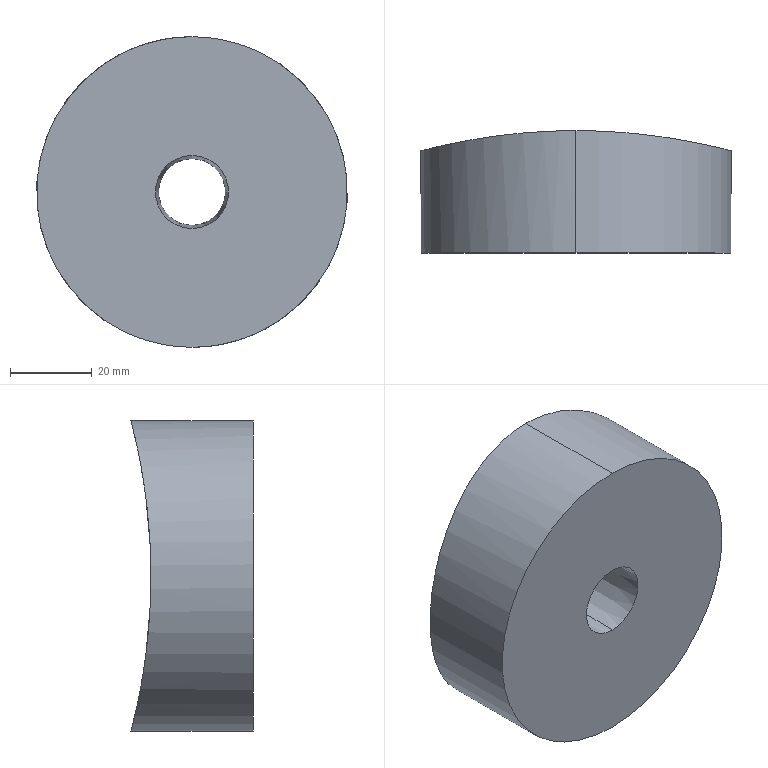Component | SolidWorks | JF21-80.1-1-3(_)-1-SOLID10-1 | 1 solid | 6 faces | box 76 x 29.89 x 76 mm | volume 113158 mm3 | cylinder 3 | cone 2 | plane 1 | commonest cylinder face diameters 76 x2 300 x1
STEP:
#1=CARTESIAN_POINT('',(-7.874,-45.267,35.9));
#2=VERTEX_POINT('',#1);
#3=CARTESIAN_POINT('',(-7.874,-45.267,36.541));
#4=VERTEX_POINT('',#3);
#5=CARTESIAN_POINT('',(-7.874,-45.267,35.9));
#6=CARTESIAN_POINT('',(-7.895,-45.267,35.9));
#7=CARTESIAN_POINT('',(-7.916,-45.267,35.902));
#8=CARTESIAN_POINT('',(-7.947,-45.267,35.908));
#9=CARTESIAN_POINT('',(-7.957,-45.267,35.91));
#10=CARTESIAN_POINT('',(-7.977,-45.268,35.916));
#11=CARTESIAN_POINT('',(-7.987,-45.268,35.92));
#12=CARTESIAN_POINT('',(-8.016,-45.269,35.932));
#13=CARTESIAN_POINT('',(-8.035,-45.269,35.942));
#14=CARTESIAN_POINT('',(-8.07,-45.27,35.965));
#15=CARTESIAN_POINT('',(-8.086,-45.271,35.979));
#16=CARTESIAN_POINT('',(-8.116,-45.272,36.008));
#17=CARTESIAN_POINT('',(-8.129,-45.272,36.024));
#18=CARTESIAN_POINT('',(-8.147,-45.273,36.051));
#19=CARTESIAN_POINT('',(-8.152,-45.273,36.06));
#20=CARTESIAN_POINT('',(-8.162,-45.274,36.078));
#21=CARTESIAN_POINT('',(-8.171,-45.274,36.097));
#22=CARTESIAN_POINT('',(-8.178,-45.275,36.117));
#23=CARTESIAN_POINT('',(-8.184,-45.275,36.137));
#24=CARTESIAN_POINT('',(-8.187,-45.275,36.147));
#25=CARTESIAN_POINT('',(-8.193,-45.275,36.178));
#26=CARTESIAN_POINT('',(-8.195,-45.276,36.199));
#27=CARTESIAN_POINT('',(-8.195,-45.276,36.231));
#28=CARTESIAN_POINT('',(-8.195,-45.276,36.241));
#29=CARTESIAN_POINT('',(-8.193,-45.275,36.262));
#30=CARTESIAN_POINT('',(-8.191,-45.275,36.273));
#31=CARTESIAN_POINT('',(-8.185,-45.275,36.304));
#32=CARTESIAN_POINT('',(-8.179,-45.275,36.324));
#33=CARTESIAN_POINT('',(-8.167,-45.274,36.353));
#34=CARTESIAN_POINT('',(-8.162,-45.274,36.362));
#35=CARTESIAN_POINT('',(-8.152,-45.273,36.381));
#36=CARTESIAN_POINT('',(-8.147,-45.273,36.39));
#37=CARTESIAN_POINT('',(-8.13,-45.272,36.416));
#38=CARTESIAN_POINT('',(-8.116,-45.272,36.432));
#39=CARTESIAN_POINT('',(-8.086,-45.271,36.462));
#40=CARTESIAN_POINT('',(-8.07,-45.27,36.476));
#41=CARTESIAN_POINT('',(-8.044,-45.269,36.493));
#42=CARTESIAN_POINT('',(-8.035,-45.269,36.498));
#43=CARTESIAN_POINT('',(-8.016,-45.269,36.508));
#44=CARTESIAN_POINT('',(-8.007,-45.268,36.513));
#45=CARTESIAN_POINT('',(-7.978,-45.268,36.525));
#46=CARTESIAN_POINT('',(-7.958,-45.267,36.531));
#47=CARTESIAN_POINT('',(-7.916,-45.267,36.539));
#48=CARTESIAN_POINT('',(-7.895,-45.267,36.541));
#49=CARTESIAN_POINT('',(-7.874,-45.267,36.541));
#50=B_SPLINE_CURVE_WITH_KNOTS('',3,(#5,#6,#7,#8,#9,#10,#11,#12,#13,#14,#15,#16,#17,#18,#19,#20,#21,#22,#23,#24,#25,#26,#27,#28,#29,#30,#31,#32,#33,#34,#35,#36,#37,#38,#39,#40,#41,#42,#43,#44,#45,#46,#47,#48,#49),.UNSPECIFIED.,.F.,.F.,(4,2,2,2,2,2,2,2,1,2,2,2,2,2,2,2,2,2,2,2,2,2,4),(0.,0.001594,0.00239,0.003187,0.004781,0.006375,0.007968,0.008765,0.009562,0.01036,0.01116,0.01275,0.01355,0.01434,0.01594,0.01673,0.01753,0.01912,0.02072,0.02151,0.02231,0.0239,0.0255),.UNSPECIFIED.);
#51=EDGE_CURVE('',#2,#4,#50,.T.);
#52=ORIENTED_EDGE('',*,*,#51,.T.);
#53=CARTESIAN_POINT('',(-7.874,-46.26,36.572));
#54=VERTEX_POINT('',#53);
#55=CARTESIAN_POINT('',(-7.874,-46.26,36.572));
#56=DIRECTION('',(-0.,0.9995,-0.0312));
#57=VECTOR('',#56,39.37);
#58=LINE('',#55,#57);
#59=EDGE_CURVE('',#54,#4,#58,.T.);
#60=ORIENTED_EDGE('',*,*,#59,.F.);
#61=CARTESIAN_POINT('',(-7.874,-46.26,35.869));
#62=VERTEX_POINT('',#61);
#63=CARTESIAN_POINT('',(-7.874,-46.26,36.22));
#64=DIRECTION('',(0.,-1.,0.));
#65=DIRECTION('',(0.,0.,-1.));
#66=AXIS2_PLACEMENT_3D('',#63,#64,#65);
#67=CIRCLE('',#66,0.352);
#68=EDGE_CURVE('',#54,#62,#67,.T.);
#69=ORIENTED_EDGE('',*,*,#68,.T.);
#70=CARTESIAN_POINT('',(-7.874,-46.26,35.869));
#71=DIRECTION('',(0.,0.9995,0.0312));
#72=VECTOR('',#71,39.37);
#73=LINE('',#70,#72);
#74=EDGE_CURVE('',#62,#2,#73,.T.);
#75=ORIENTED_EDGE('',*,*,#74,.T.);
#76=EDGE_LOOP('',(#52,#60,#69,#75));
#77=FACE_OUTER_BOUND('',#76,.T.);
#78=CARTESIAN_POINT('',(-7.874,-46.26,36.22));
#79=DIRECTION('',(0.,-1.,0.));
#80=DIRECTION('',(0.,0.,1.));
#81=AXIS2_PLACEMENT_3D('',#78,#79,#80);
#82=CONICAL_SURFACE('',#81,0.352,0.03121);
#83=ADVANCED_FACE('',(#77),#82,.F.);
#84=CARTESIAN_POINT('',(-7.874,-45.083,37.717));
#85=VERTEX_POINT('',#84);
#86=CARTESIAN_POINT('',(-7.874,-45.083,34.724));
#87=VERTEX_POINT('',#86);
#88=CARTESIAN_POINT('',(-7.874,-45.083,37.717));
#89=CARTESIAN_POINT('',(-7.775,-45.083,37.717));
#90=CARTESIAN_POINT('',(-7.677,-45.086,37.707));
#91=CARTESIAN_POINT('',(-7.533,-45.093,37.678));
#92=CARTESIAN_POINT('',(-7.486,-45.096,37.666));
#93=CARTESIAN_POINT('',(-7.415,-45.101,37.645));
#94=CARTESIAN_POINT('',(-7.392,-45.103,37.637));
#95=CARTESIAN_POINT('',(-7.345,-45.107,37.62));
#96=CARTESIAN_POINT('',(-7.322,-45.109,37.611));
#97=CARTESIAN_POINT('',(-7.209,-45.121,37.564));
#98=CARTESIAN_POINT('',(-7.124,-45.131,37.518));
#99=CARTESIAN_POINT('',(-7.022,-45.146,37.451));
#100=CARTESIAN_POINT('',(-7.002,-45.149,37.437));
#101=CARTESIAN_POINT('',(-6.963,-45.155,37.407));
#102=CARTESIAN_POINT('',(-6.943,-45.158,37.392));
#103=CARTESIAN_POINT('',(-6.887,-45.168,37.345));
#104=CARTESIAN_POINT('',(-6.85,-45.174,37.313));
#105=CARTESIAN_POINT('',(-6.747,-45.193,37.21));
#106=CARTESIAN_POINT('',(-6.686,-45.205,37.135));
#107=CARTESIAN_POINT('',(-6.617,-45.22,37.033));
#108=CARTESIAN_POINT('',(-6.604,-45.222,37.012));
#109=CARTESIAN_POINT('',(-6.579,-45.228,36.97));
#110=CARTESIAN_POINT('',(-6.567,-45.231,36.948));
#111=CARTESIAN_POINT('',(-6.532,-45.238,36.884));
#112=CARTESIAN_POINT('',(-6.511,-45.243,36.84));
#113=CARTESIAN_POINT('',(-6.474,-45.252,36.75));
#114=CARTESIAN_POINT('',(-6.457,-45.256,36.704));
#115=CARTESIAN_POINT('',(-6.436,-45.261,36.634));
#116=CARTESIAN_POINT('',(-6.429,-45.263,36.61));
#117=CARTESIAN_POINT('',(-6.417,-45.266,36.562));
#118=CARTESIAN_POINT('',(-6.412,-45.267,36.538));
#119=CARTESIAN_POINT('',(-6.388,-45.273,36.417));
#120=CARTESIAN_POINT('',(-6.378,-45.276,36.32));
#121=CARTESIAN_POINT('',(-6.378,-45.276,36.173));
#122=CARTESIAN_POINT('',(-6.38,-45.275,36.124));
#123=CARTESIAN_POINT('',(-6.39,-45.273,36.025));
#124=CARTESIAN_POINT('',(-6.397,-45.271,35.976));
#125=CARTESIAN_POINT('',(-6.426,-45.264,35.832));
#126=CARTESIAN_POINT('',(-6.454,-45.257,35.739));
#127=CARTESIAN_POINT('',(-6.501,-45.246,35.625));
#128=CARTESIAN_POINT('',(-6.511,-45.243,35.602));
#129=CARTESIAN_POINT('',(-6.532,-45.238,35.558));
#130=CARTESIAN_POINT('',(-6.543,-45.236,35.536));
#131=CARTESIAN_POINT('',(-6.578,-45.228,35.471));
#132=CARTESIAN_POINT('',(-6.603,-45.223,35.43));
#133=CARTESIAN_POINT('',(-6.657,-45.211,35.349));
#134=CARTESIAN_POINT('',(-6.686,-45.205,35.31));
#135=CARTESIAN_POINT('',(-6.733,-45.196,35.253));
#136=CARTESIAN_POINT('',(-6.748,-45.193,35.235));
#137=CARTESIAN_POINT('',(-6.781,-45.186,35.198));
#138=CARTESIAN_POINT('',(-6.798,-45.183,35.18));
#139=CARTESIAN_POINT('',(-6.885,-45.168,35.094));
#140=CARTESIAN_POINT('',(-6.96,-45.155,35.032));
#141=CARTESIAN_POINT('',(-7.081,-45.138,34.951));
#142=CARTESIAN_POINT('',(-7.123,-45.132,34.926));
#143=CARTESIAN_POINT('',(-7.188,-45.124,34.891));
#144=CARTESIAN_POINT('',(-7.21,-45.121,34.88));
#145=CARTESIAN_POINT('',(-7.254,-45.116,34.859));
#146=CARTESIAN_POINT('',(-7.277,-45.114,34.849));
#147=CARTESIAN_POINT('',(-7.39,-45.103,34.802));
#148=CARTESIAN_POINT('',(-7.483,-45.096,34.773));
#149=CARTESIAN_POINT('',(-7.603,-45.089,34.749));
#150=CARTESIAN_POINT('',(-7.627,-45.088,34.745));
#151=CARTESIAN_POINT('',(-7.676,-45.086,34.737));
#152=CARTESIAN_POINT('',(-7.701,-45.086,34.734));
#153=CARTESIAN_POINT('',(-7.775,-45.084,34.727));
#154=CARTESIAN_POINT('',(-7.824,-45.083,34.724));
#155=CARTESIAN_POINT('',(-7.874,-45.083,34.724));
#156=B_SPLINE_CURVE_WITH_KNOTS('',3,(#88,#89,#90,#91,#92,#93,#94,#95,#96,#97,#98,#99,#100,#101,#102,#103,#104,#105,#106,#107,#108,#109,#110,#111,#112,#113,#114,#115,#116,#117,#118,#119,#120,#121,#122,#123,#124,#125,#126,#127,#128,#129,#130,#131,#132,#133,#134,#135,#136,#137,#138,#139,#140,#141,#142,#143,#144,#145,#146,#147,#148,#149,#150,#151,#152,#153,#154,#155),.UNSPECIFIED.,.F.,.F.,(4,2,2,2,2,2,2,2,2,2,2,2,2,2,2,2,2,2,2,2,2,2,2,2,2,2,2,2,2,2,2,2,2,4),(0.,0.007453,0.01118,0.01304,0.01491,0.02236,0.02422,0.02609,0.02981,0.03727,0.03913,0.04099,0.04472,0.04845,0.05031,0.05217,0.05963,0.06335,0.06708,0.07453,0.0764,0.07826,0.08199,0.08571,0.08758,0.08944,0.09689,0.1006,0.1025,0.1043,0.1118,0.1137,0.1155,0.1193),.UNSPECIFIED.);
#157=EDGE_CURVE('',#85,#87,#156,.T.);
#158=ORIENTED_EDGE('',*,*,#157,.F.);
#159=CARTESIAN_POINT('',(-7.874,-46.26,37.717));
#160=VERTEX_POINT('',#159);
#161=CARTESIAN_POINT('',(-7.874,-44.882,37.717));
#162=DIRECTION('',(0.,1.,0.));
#163=VECTOR('',#162,39.37);
#164=LINE('',#161,#163);
#165=EDGE_CURVE('',#160,#85,#164,.T.);
#166=ORIENTED_EDGE('',*,*,#165,.F.);
#167=CARTESIAN_POINT('',(-7.874,-46.26,34.724));
#168=VERTEX_POINT('',#167);
#169=CARTESIAN_POINT('',(-7.874,-46.26,36.22));
#170=DIRECTION('',(0.,1.,0.));
#171=DIRECTION('',(0.,0.,1.));
#172=AXIS2_PLACEMENT_3D('',#169,#170,#171);
#173=CIRCLE('',#172,1.496);
#174=EDGE_CURVE('',#160,#168,#173,.T.);
#175=ORIENTED_EDGE('',*,*,#174,.T.);
#176=CARTESIAN_POINT('',(-7.874,-44.882,34.724));
#177=DIRECTION('',(0.,1.,0.));
#178=VECTOR('',#177,39.37);
#179=LINE('',#176,#178);
#180=EDGE_CURVE('',#168,#87,#179,.T.);
#181=ORIENTED_EDGE('',*,*,#180,.T.);
#182=EDGE_LOOP('',(#158,#166,#175,#181));
#183=FACE_OUTER_BOUND('',#182,.T.);
#184=CARTESIAN_POINT('',(-7.874,-44.882,36.22));
#185=DIRECTION('',(0.,-1.,0.));
#186=DIRECTION('',(0.,0.,1.));
#187=AXIS2_PLACEMENT_3D('',#184,#185,#186);
#188=CYLINDRICAL_SURFACE('',#187,1.496);
#189=ADVANCED_FACE('',(#183),#188,.T.);
#190=ORIENTED_EDGE('',*,*,#165,.T.);
#191=CARTESIAN_POINT('',(-7.874,-45.083,34.724));
#192=CARTESIAN_POINT('',(-7.973,-45.083,34.724));
#193=CARTESIAN_POINT('',(-8.071,-45.086,34.734));
#194=CARTESIAN_POINT('',(-8.215,-45.093,34.763));
#195=CARTESIAN_POINT('',(-8.262,-45.096,34.775));
#196=CARTESIAN_POINT('',(-8.333,-45.101,34.796));
#197=CARTESIAN_POINT('',(-8.356,-45.103,34.804));
#198=CARTESIAN_POINT('',(-8.403,-45.107,34.821));
#199=CARTESIAN_POINT('',(-8.426,-45.109,34.83));
#200=CARTESIAN_POINT('',(-8.539,-45.121,34.877));
#201=CARTESIAN_POINT('',(-8.624,-45.131,34.923));
#202=CARTESIAN_POINT('',(-8.726,-45.146,34.99));
#203=CARTESIAN_POINT('',(-8.746,-45.149,35.004));
#204=CARTESIAN_POINT('',(-8.785,-45.155,35.034));
#205=CARTESIAN_POINT('',(-8.805,-45.158,35.049));
#206=CARTESIAN_POINT('',(-8.861,-45.168,35.095));
#207=CARTESIAN_POINT('',(-8.898,-45.174,35.128));
#208=CARTESIAN_POINT('',(-9.001,-45.193,35.231));
#209=CARTESIAN_POINT('',(-9.062,-45.205,35.306));
#210=CARTESIAN_POINT('',(-9.131,-45.22,35.408));
#211=CARTESIAN_POINT('',(-9.144,-45.222,35.429));
#212=CARTESIAN_POINT('',(-9.169,-45.228,35.471));
#213=CARTESIAN_POINT('',(-9.181,-45.231,35.492));
#214=CARTESIAN_POINT('',(-9.216,-45.238,35.557));
#215=CARTESIAN_POINT('',(-9.237,-45.243,35.601));
#216=CARTESIAN_POINT('',(-9.274,-45.252,35.691));
#217=CARTESIAN_POINT('',(-9.291,-45.256,35.737));
#218=CARTESIAN_POINT('',(-9.312,-45.261,35.807));
#219=CARTESIAN_POINT('',(-9.319,-45.263,35.831));
#220=CARTESIAN_POINT('',(-9.331,-45.266,35.879));
#221=CARTESIAN_POINT('',(-9.336,-45.267,35.903));
#222=CARTESIAN_POINT('',(-9.36,-45.273,36.024));
#223=CARTESIAN_POINT('',(-9.37,-45.276,36.121));
#224=CARTESIAN_POINT('',(-9.37,-45.276,36.268));
#225=CARTESIAN_POINT('',(-9.368,-45.275,36.317));
#226=CARTESIAN_POINT('',(-9.358,-45.273,36.416));
#227=CARTESIAN_POINT('',(-9.351,-45.271,36.465));
#228=CARTESIAN_POINT('',(-9.322,-45.264,36.609));
#229=CARTESIAN_POINT('',(-9.294,-45.257,36.702));
#230=CARTESIAN_POINT('',(-9.247,-45.246,36.816));
#231=CARTESIAN_POINT('',(-9.237,-45.243,36.838));
#232=CARTESIAN_POINT('',(-9.216,-45.238,36.883));
#233=CARTESIAN_POINT('',(-9.205,-45.236,36.905));
#234=CARTESIAN_POINT('',(-9.17,-45.228,36.97));
#235=CARTESIAN_POINT('',(-9.145,-45.223,37.011));
#236=CARTESIAN_POINT('',(-9.091,-45.211,37.092));
#237=CARTESIAN_POINT('',(-9.062,-45.205,37.131));
#238=CARTESIAN_POINT('',(-9.016,-45.196,37.188));
#239=CARTESIAN_POINT('',(-9.,-45.193,37.206));
#240=CARTESIAN_POINT('',(-8.967,-45.186,37.243));
#241=CARTESIAN_POINT('',(-8.95,-45.183,37.261));
#242=CARTESIAN_POINT('',(-8.863,-45.168,37.347));
#243=CARTESIAN_POINT('',(-8.788,-45.155,37.409));
#244=CARTESIAN_POINT('',(-8.667,-45.138,37.49));
#245=CARTESIAN_POINT('',(-8.625,-45.132,37.515));
#246=CARTESIAN_POINT('',(-8.56,-45.124,37.55));
#247=CARTESIAN_POINT('',(-8.538,-45.121,37.561));
#248=CARTESIAN_POINT('',(-8.494,-45.116,37.582));
#249=CARTESIAN_POINT('',(-8.471,-45.114,37.592));
#250=CARTESIAN_POINT('',(-8.358,-45.103,37.639));
#251=CARTESIAN_POINT('',(-8.265,-45.096,37.668));
#252=CARTESIAN_POINT('',(-8.145,-45.089,37.692));
#253=CARTESIAN_POINT('',(-8.121,-45.088,37.696));
#254=CARTESIAN_POINT('',(-8.072,-45.086,37.704));
#255=CARTESIAN_POINT('',(-8.047,-45.086,37.707));
#256=CARTESIAN_POINT('',(-7.973,-45.084,37.714));
#257=CARTESIAN_POINT('',(-7.924,-45.083,37.717));
#258=CARTESIAN_POINT('',(-7.874,-45.083,37.717));
#259=B_SPLINE_CURVE_WITH_KNOTS('',3,(#191,#192,#193,#194,#195,#196,#197,#198,#199,#200,#201,#202,#203,#204,#205,#206,#207,#208,#209,#210,#211,#212,#213,#214,#215,#216,#217,#218,#219,#220,#221,#222,#223,#224,#225,#226,#227,#228,#229,#230,#231,#232,#233,#234,#235,#236,#237,#238,#239,#240,#241,#242,#243,#244,#245,#246,#247,#248,#249,#250,#251,#252,#253,#254,#255,#256,#257,#258),.UNSPECIFIED.,.F.,.F.,(4,2,2,2,2,2,2,2,2,2,2,2,2,2,2,2,2,2,2,2,2,2,2,2,2,2,2,2,2,2,2,2,2,4),(0.,0.007453,0.01118,0.01304,0.01491,0.02236,0.02422,0.02609,0.02981,0.03727,0.03913,0.04099,0.04472,0.04845,0.05031,0.05217,0.05963,0.06335,0.06708,0.07453,0.0764,0.07826,0.08199,0.08571,0.08758,0.08944,0.09689,0.1006,0.1025,0.1043,0.1118,0.1137,0.1155,0.1193),.UNSPECIFIED.);
#260=EDGE_CURVE('',#87,#85,#259,.T.);
#261=ORIENTED_EDGE('',*,*,#260,.F.);
#262=ORIENTED_EDGE('',*,*,#180,.F.);
#263=CARTESIAN_POINT('',(-7.874,-46.26,36.22));
#264=DIRECTION('',(0.,1.,0.));
#265=DIRECTION('',(0.,0.,1.));
#266=AXIS2_PLACEMENT_3D('',#263,#264,#265);
#267=CIRCLE('',#266,1.496);
#268=EDGE_CURVE('',#168,#160,#267,.T.);
#269=ORIENTED_EDGE('',*,*,#268,.T.);
#270=EDGE_LOOP('',(#190,#261,#262,#269));
#271=FACE_OUTER_BOUND('',#270,.T.);
#272=CARTESIAN_POINT('',(-7.874,-44.882,36.22));
#273=DIRECTION('',(0.,-1.,0.));
#274=DIRECTION('',(0.,0.,1.));
#275=AXIS2_PLACEMENT_3D('',#272,#273,#274);
#276=CYLINDRICAL_SURFACE('',#275,1.496);
#277=ADVANCED_FACE('',(#271),#276,.T.);
#278=CARTESIAN_POINT('',(-7.874,-46.26,36.22));
#279=DIRECTION('',(0.,-1.,0.));
#280=DIRECTION('',(0.,0.,-1.));
#281=AXIS2_PLACEMENT_3D('',#278,#279,#280);
#282=CIRCLE('',#281,0.352);
#283=EDGE_CURVE('',#62,#54,#282,.T.);
#284=ORIENTED_EDGE('',*,*,#283,.F.);
#285=ORIENTED_EDGE('',*,*,#68,.F.);
#286=EDGE_LOOP('',(#284,#285));
#287=FACE_BOUND('',#286,.T.);
#288=ORIENTED_EDGE('',*,*,#268,.F.);
#289=ORIENTED_EDGE('',*,*,#174,.F.);
#290=EDGE_LOOP('',(#288,#289));
#291=FACE_OUTER_BOUND('',#290,.T.);
#292=CARTESIAN_POINT('',(-7.874,-46.26,36.22));
#293=DIRECTION('',(0.,1.,0.));
#294=DIRECTION('',(0.,0.,-1.));
#295=AXIS2_PLACEMENT_3D('',#292,#293,#294);
#296=PLANE('',#295);
#297=ADVANCED_FACE('',(#287,#291),#296,.F.);
#298=ORIENTED_EDGE('',*,*,#51,.F.);
#299=CARTESIAN_POINT('',(-7.874,-45.267,36.541));
#300=CARTESIAN_POINT('',(-7.853,-45.267,36.541));
#301=CARTESIAN_POINT('',(-7.832,-45.267,36.539));
#302=CARTESIAN_POINT('',(-7.801,-45.267,36.533));
#303=CARTESIAN_POINT('',(-7.791,-45.267,36.531));
#304=CARTESIAN_POINT('',(-7.771,-45.268,36.525));
#305=CARTESIAN_POINT('',(-7.761,-45.268,36.521));
#306=CARTESIAN_POINT('',(-7.732,-45.269,36.509));
#307=CARTESIAN_POINT('',(-7.713,-45.269,36.499));
#308=CARTESIAN_POINT('',(-7.678,-45.27,36.476));
#309=CARTESIAN_POINT('',(-7.662,-45.271,36.462));
#310=CARTESIAN_POINT('',(-7.632,-45.272,36.433));
#311=CARTESIAN_POINT('',(-7.619,-45.272,36.417));
#312=CARTESIAN_POINT('',(-7.601,-45.273,36.39));
#313=CARTESIAN_POINT('',(-7.596,-45.273,36.381));
#314=CARTESIAN_POINT('',(-7.586,-45.274,36.363));
#315=CARTESIAN_POINT('',(-7.577,-45.274,36.344));
#316=CARTESIAN_POINT('',(-7.57,-45.275,36.324));
#317=CARTESIAN_POINT('',(-7.564,-45.275,36.304));
#318=CARTESIAN_POINT('',(-7.561,-45.275,36.294));
#319=CARTESIAN_POINT('',(-7.555,-45.275,36.262));
#320=CARTESIAN_POINT('',(-7.553,-45.276,36.242));
#321=CARTESIAN_POINT('',(-7.553,-45.276,36.21));
#322=CARTESIAN_POINT('',(-7.553,-45.276,36.2));
#323=CARTESIAN_POINT('',(-7.555,-45.275,36.179));
#324=CARTESIAN_POINT('',(-7.557,-45.275,36.168));
#325=CARTESIAN_POINT('',(-7.563,-45.275,36.137));
#326=CARTESIAN_POINT('',(-7.569,-45.275,36.117));
#327=CARTESIAN_POINT('',(-7.581,-45.274,36.088));
#328=CARTESIAN_POINT('',(-7.586,-45.274,36.079));
#329=CARTESIAN_POINT('',(-7.596,-45.273,36.06));
#330=CARTESIAN_POINT('',(-7.601,-45.273,36.051));
#331=CARTESIAN_POINT('',(-7.618,-45.272,36.025));
#332=CARTESIAN_POINT('',(-7.632,-45.272,36.009));
#333=CARTESIAN_POINT('',(-7.662,-45.271,35.979));
#334=CARTESIAN_POINT('',(-7.678,-45.27,35.965));
#335=CARTESIAN_POINT('',(-7.704,-45.269,35.948));
#336=CARTESIAN_POINT('',(-7.713,-45.269,35.943));
#337=CARTESIAN_POINT('',(-7.732,-45.269,35.933));
#338=CARTESIAN_POINT('',(-7.741,-45.268,35.928));
#339=CARTESIAN_POINT('',(-7.77,-45.268,35.916));
#340=CARTESIAN_POINT('',(-7.79,-45.267,35.91));
#341=CARTESIAN_POINT('',(-7.832,-45.267,35.902));
#342=CARTESIAN_POINT('',(-7.853,-45.267,35.9));
#343=CARTESIAN_POINT('',(-7.874,-45.267,35.9));
#344=B_SPLINE_CURVE_WITH_KNOTS('',3,(#299,#300,#301,#302,#303,#304,#305,#306,#307,#308,#309,#310,#311,#312,#313,#314,#315,#316,#317,#318,#319,#320,#321,#322,#323,#324,#325,#326,#327,#328,#329,#330,#331,#332,#333,#334,#335,#336,#337,#338,#339,#340,#341,#342,#343),.UNSPECIFIED.,.F.,.F.,(4,2,2,2,2,2,2,2,1,2,2,2,2,2,2,2,2,2,2,2,2,2,4),(0.,0.001594,0.00239,0.003187,0.004781,0.006375,0.007968,0.008765,0.009562,0.01036,0.01116,0.01275,0.01355,0.01434,0.01594,0.01673,0.01753,0.01912,0.02072,0.02151,0.02231,0.0239,0.0255),.UNSPECIFIED.);
#345=EDGE_CURVE('',#4,#2,#344,.T.);
#346=ORIENTED_EDGE('',*,*,#345,.F.);
#347=EDGE_LOOP('',(#298,#346));
#348=FACE_BOUND('',#347,.T.);
#349=ORIENTED_EDGE('',*,*,#260,.T.);
#350=ORIENTED_EDGE('',*,*,#157,.T.);
#351=EDGE_LOOP('',(#349,#350));
#352=FACE_OUTER_BOUND('',#351,.T.);
#353=CARTESIAN_POINT('',(-15.748,-39.37,36.22));
#354=DIRECTION('',(1.,0.,0.));
#355=DIRECTION('',(0.,0.,1.));
#356=AXIS2_PLACEMENT_3D('',#353,#354,#355);
#357=CYLINDRICAL_SURFACE('',#356,5.906);
#358=ADVANCED_FACE('',(#348,#352),#357,.F.);
#359=ORIENTED_EDGE('',*,*,#59,.T.);
#360=ORIENTED_EDGE('',*,*,#345,.T.);
#361=ORIENTED_EDGE('',*,*,#74,.F.);
#362=ORIENTED_EDGE('',*,*,#283,.T.);
#363=EDGE_LOOP('',(#359,#360,#361,#362));
#364=FACE_OUTER_BOUND('',#363,.T.);
#365=CARTESIAN_POINT('',(-7.874,-46.26,36.22));
#366=DIRECTION('',(0.,-1.,0.));
#367=DIRECTION('',(0.,0.,1.));
#368=AXIS2_PLACEMENT_3D('',#365,#366,#367);
#369=CONICAL_SURFACE('',#368,0.352,0.03121);
#370=ADVANCED_FACE('',(#364),#369,.F.);
#371=CLOSED_SHELL('',(#83,#189,#277,#297,#358,#370));
#372=MANIFOLD_SOLID_BREP('',#371);
#373=CARTESIAN_POINT('',(0.,0.,0.));
#374=DIRECTION('',(0.,0.,1.));
#375=DIRECTION('',(1.,0.,0.));
#376=AXIS2_PLACEMENT_3D('',#373,#374,#375);
#377=(LENGTH_UNIT()NAMED_UNIT(*)SI_UNIT($,.METRE.));
#378=LENGTH_MEASURE_WITH_UNIT(LENGTH_MEASURE(0.0254),#377);
#379=DIMENSIONAL_EXPONENTS(1.,0.,0.,0.,0.,0.,0.);
#380=(CONVERSION_BASED_UNIT('',#378)LENGTH_UNIT()NAMED_UNIT(#379));
#381=UNCERTAINTY_MEASURE_WITH_UNIT(LENGTH_MEASURE(0.00001),#380,'','');
#382=(NAMED_UNIT(*)PLANE_ANGLE_UNIT()SI_UNIT($,.RADIAN.));
#383=(NAMED_UNIT(*)SI_UNIT($,.STERADIAN.)SOLID_ANGLE_UNIT());
#384=(GEOMETRIC_REPRESENTATION_CONTEXT(3)GLOBAL_UNCERTAINTY_ASSIGNED_CONTEXT((#381))GLOBAL_UNIT_ASSIGNED_CONTEXT((#380,#382,#383))REPRESENTATION_CONTEXT('',''));
#385=ADVANCED_BREP_SHAPE_REPRESENTATION('',(#372,#376),#384);
#386=COLOUR_RGB('',0.7922,0.8196,0.9333);
#387=FILL_AREA_STYLE_COLOUR('',#386);
#388=FILL_AREA_STYLE('',(#387));
#389=SURFACE_STYLE_FILL_AREA(#388);
#390=SURFACE_SIDE_STYLE('',(#389));
#391=SURFACE_STYLE_USAGE(.BOTH.,#390);
#392=PRESENTATION_STYLE_ASSIGNMENT((#391));
#393=STYLED_ITEM('',(#392),#372);
#394=(LENGTH_UNIT()NAMED_UNIT(*)SI_UNIT($,.METRE.));
#395=LENGTH_MEASURE_WITH_UNIT(LENGTH_MEASURE(0.0254),#394);
#396=DIMENSIONAL_EXPONENTS(1.,0.,0.,0.,0.,0.,0.);
#397=(CONVERSION_BASED_UNIT('',#395)LENGTH_UNIT()NAMED_UNIT(#396));
#398=UNCERTAINTY_MEASURE_WITH_UNIT(LENGTH_MEASURE(0.00001),#397,'','');
#399=(NAMED_UNIT(*)PLANE_ANGLE_UNIT()SI_UNIT($,.RADIAN.));
#400=(NAMED_UNIT(*)SI_UNIT($,.STERADIAN.)SOLID_ANGLE_UNIT());
#401=(GEOMETRIC_REPRESENTATION_CONTEXT(3)GLOBAL_UNCERTAINTY_ASSIGNED_CONTEXT((#398))GLOBAL_UNIT_ASSIGNED_CONTEXT((#397,#399,#400))REPRESENTATION_CONTEXT('',''));
#402=MECHANICAL_DESIGN_GEOMETRIC_PRESENTATION_REPRESENTATION('',(#393),#401);
#403=PRESENTATION_LAYER_ASSIGNMENT('','',(#393));